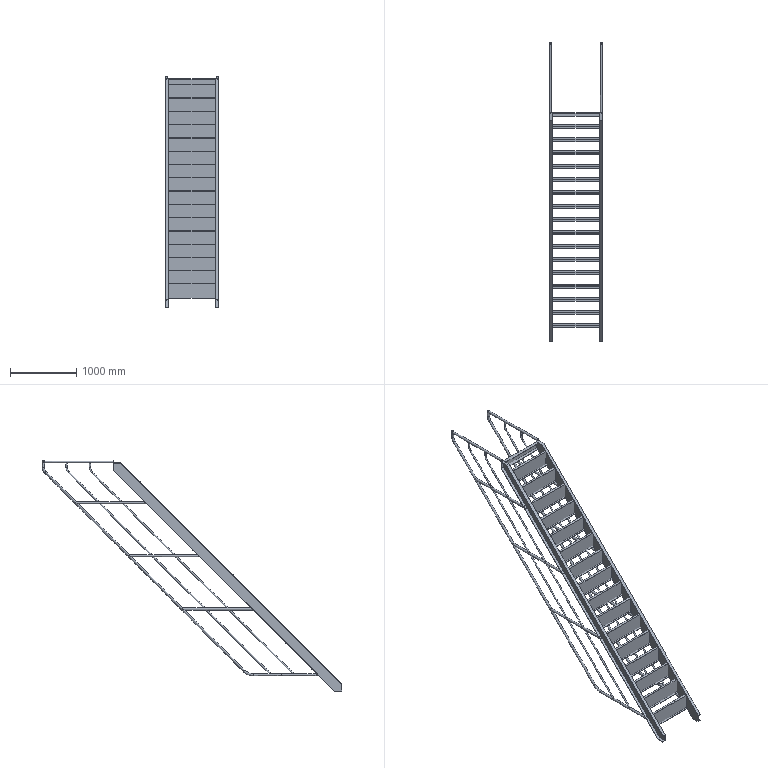Component | NX | F6 | 21 solids | 258 faces | volume 43739087 mm3 | plane 212 | spline 36 | cylinder 8 | other 2 | commonest cylinder face diameters 33.5 x8